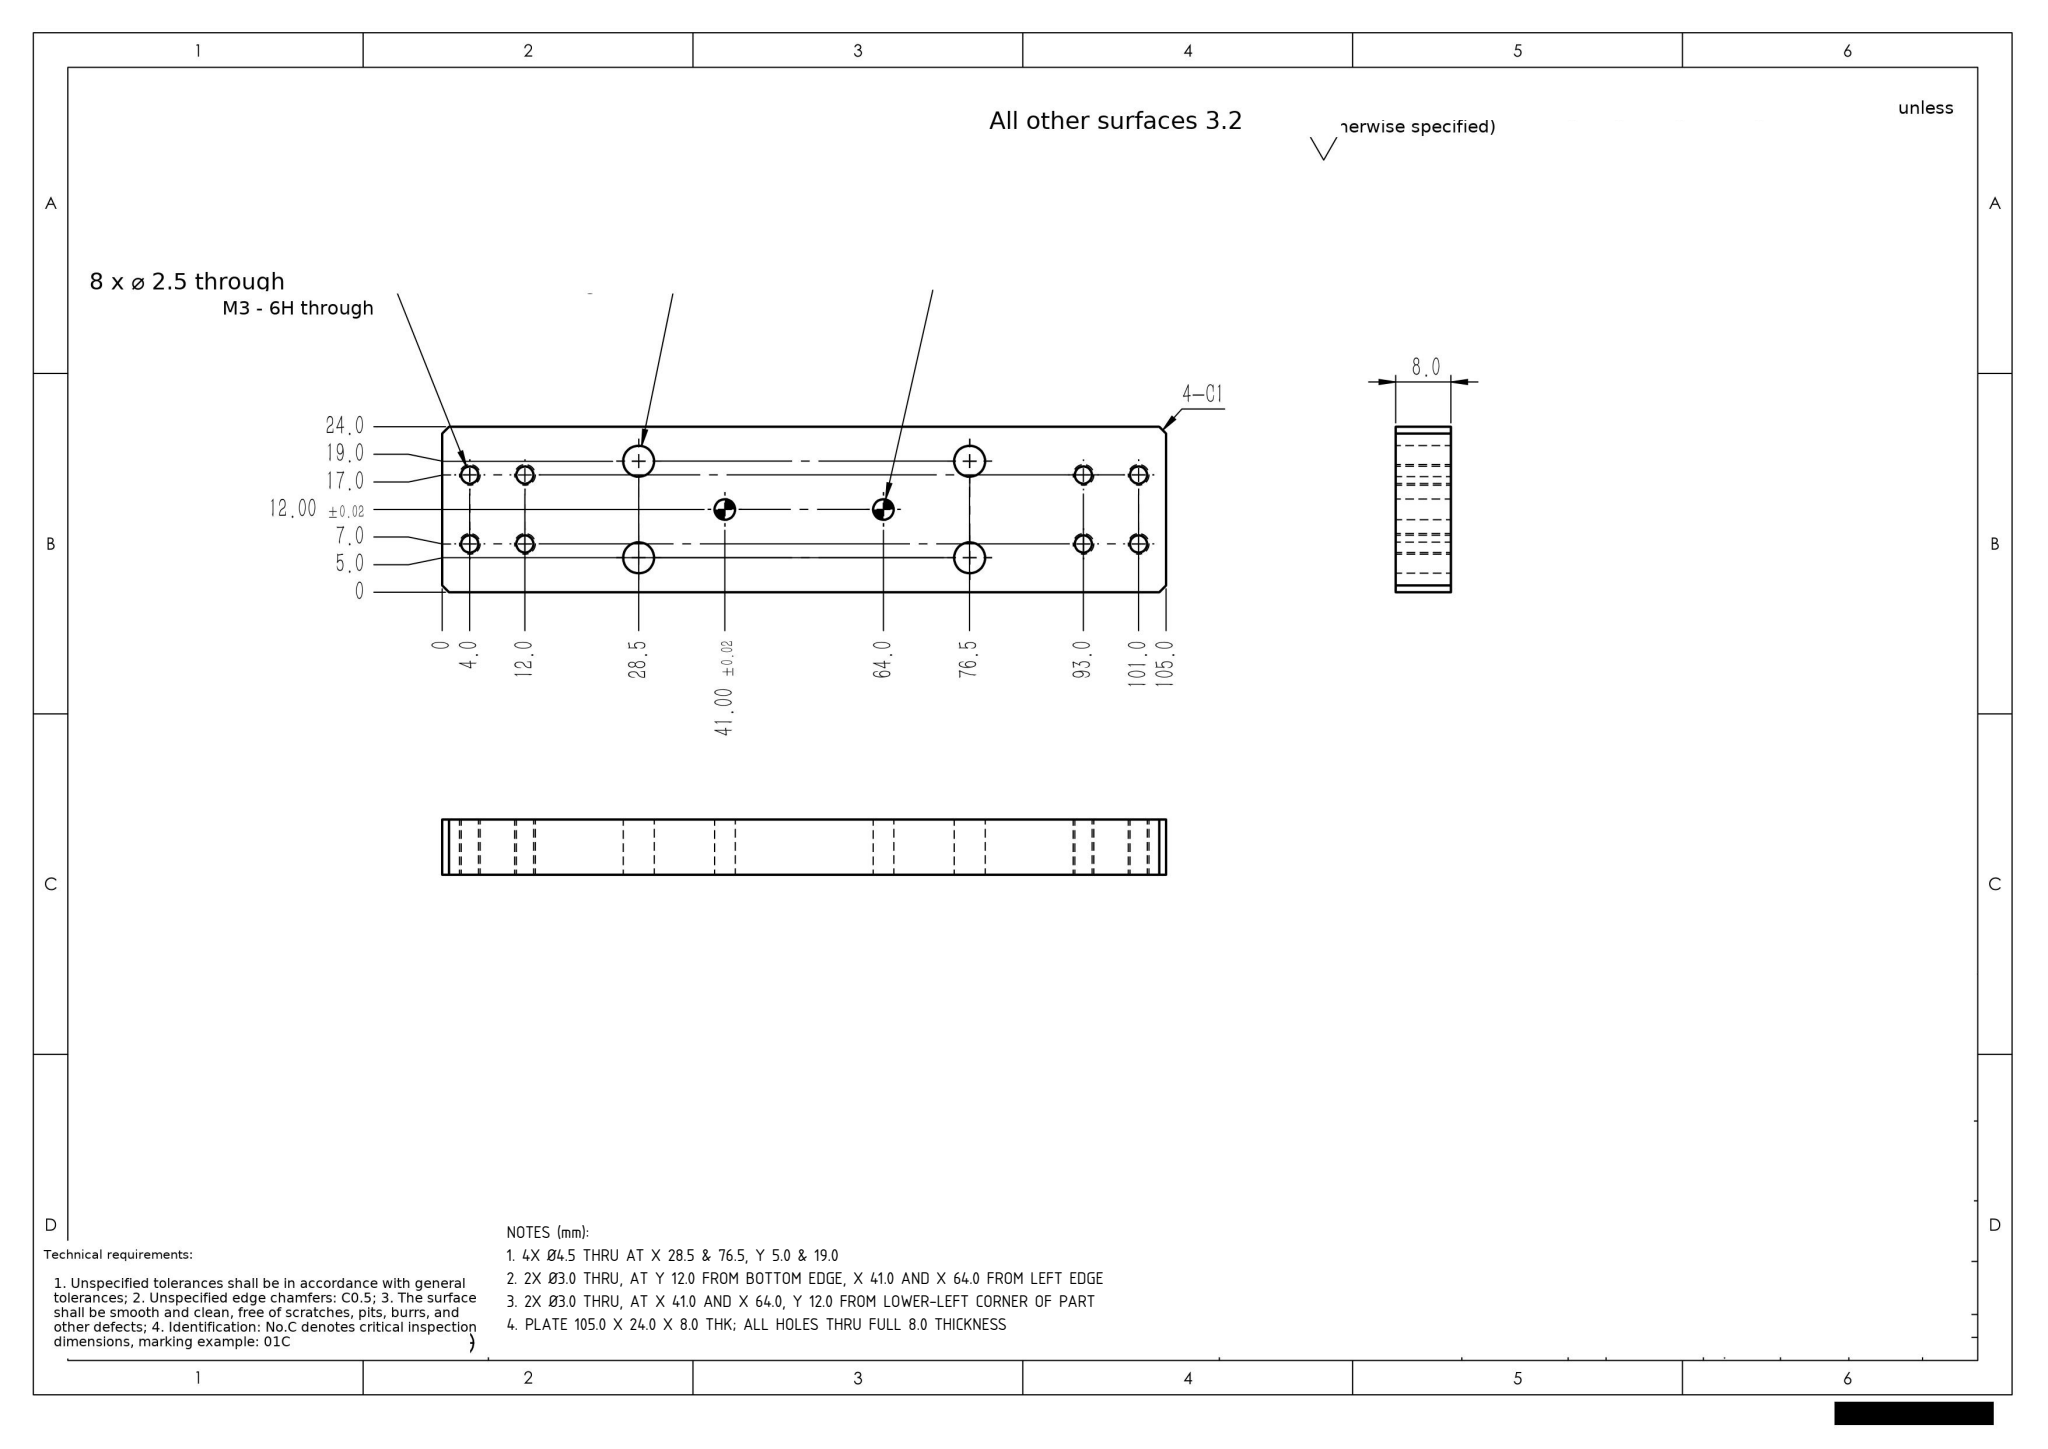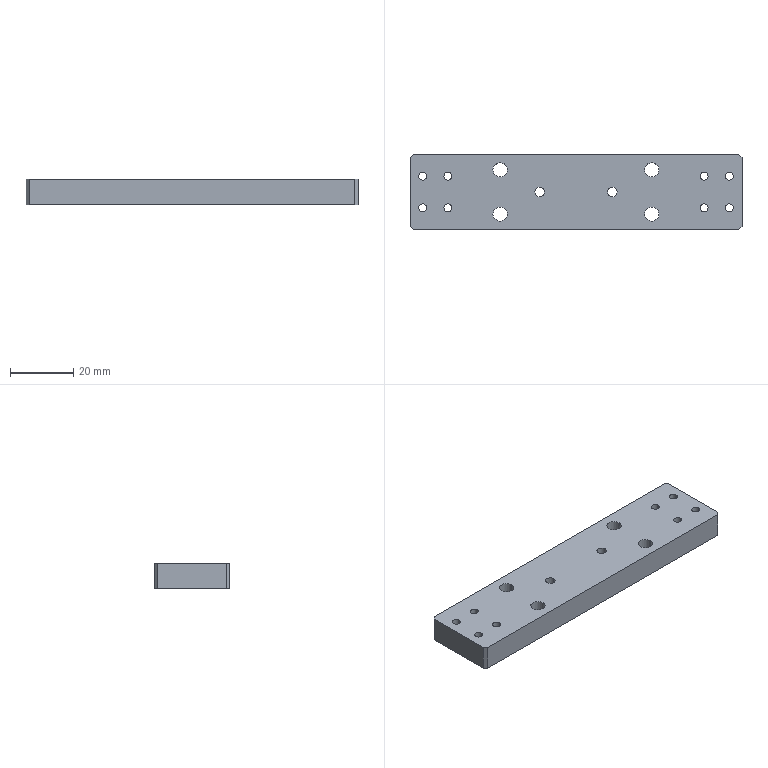Part | SolidWorks | mm | 1 solid | 38 faces | box 105 x 24 x 8 mm | volume 19208 mm3 | cylinder 28 | plane 10 | commonest cylinder face diameters 2.5 x16 4.5 x8 3 x4
Drawing notes:
4X Ø4.5 THRU AT X 28.5 & 76.5, Y 5.0 & 19.0 | from the solid: cylinders dia 4.5, axis z, pos (28.5,5.0),(28.5,19.0),(76.5,5.0),(76.5,19.0), length 8.0 = full thickness
2X Ø3.0 THRU, AT Y 12.0 FROM BOTTOM EDGE, X 41.0 AND X 64.0 FROM LEFT EDGE | from the solid: cylinders dia 3.0, axis z, pos [41.0,12.0] and [64.0,12.0], length 8.0 (full 8.0 plate thickness)
2X Ø3.0 THRU, AT X 41.0 AND X 64.0, Y 12.0 FROM LOWER-LEFT CORNER OF PART | from the solid: cylinders dia 3.0 axis z at [41.0,12.0] and [64.0,12.0], length 8.0 (full 8.0 thickness)
PLATE 105.0 X 24.0 X 8.0 THK; ALL HOLES THRU FULL 8.0 THICKNESS | from the solid: bbox_xyz [105.0,24.0,8.0]; axis_planes z 0.0 and z 8.0; all cylinder lengths 8.0
build123d program:
from build123d import *

# Parameters (mm, degrees)
SKETCH1_W            = 105
SKETCH1_H            = 24
BOSS_EXTRUDE1_DEPTH  = 8
CHAMFER1_SIZE        = 1
M4_CLEARANCE_HOLE1_D = 4.5
SKETCH6_R            = 1.5
CUT_EXTRUDE1_DEPTH   = 55.445
M3_TAPPED_HOLE1_D    = 2.5


with BuildPart() as part:
    # Sketch1 → Boss-Extrude1 (new body)
    with BuildSketch(Plane.XY):
        Rectangle(SKETCH1_W, SKETCH1_H)
    extrude(amount=BOSS_EXTRUDE1_DEPTH)

    # Chamfer1
    chamfer1_edges = [part.edges().sort_by_distance(p)[0] for p in [
        (-52.5, 12, 4),
        (52.5, 12, 4),
        (52.5, -12, 4),
        (-52.5, -12, 4),
    ]]
    chamfer(chamfer1_edges, length=CHAMFER1_SIZE)

    # M4 Clearance Hole1 (through all)
    with Locations(Plane(origin=(0, 0, 0), x_dir=(-1, 0, 0), z_dir=(0, 0, -1))):
        with Locations((-24, 7), (24, 7), (24, -7), (-24, -7)):
            Hole(M4_CLEARANCE_HOLE1_D / 2)

    # Sketch6 → Cut-Extrude1 (cut, through all)
    with BuildSketch(Plane(origin=(0, 0, 0), x_dir=(-1, 0, 0), z_dir=(0, 0, -1))):
        with Locations((-11.5, 0)):
            Circle(SKETCH6_R)
        with Locations((11.5, 0)):
            Circle(SKETCH6_R)
    extrude(amount=-CUT_EXTRUDE1_DEPTH, mode=Mode.SUBTRACT)

    # M3 Tapped Hole1 (through all)
    with Locations(Plane(origin=(0, 0, 0), x_dir=(-1, 0, 0), z_dir=(0, 0, -1))):
        with Locations((40.5, 5), (48.5, 5), (48.5, -5), (40.5, -5), (-40.5, 5), (-40.5, -5), (-48.5, -5), (-48.5, 5)):
            Hole(M3_TAPPED_HOLE1_D / 2)


solid = part.part